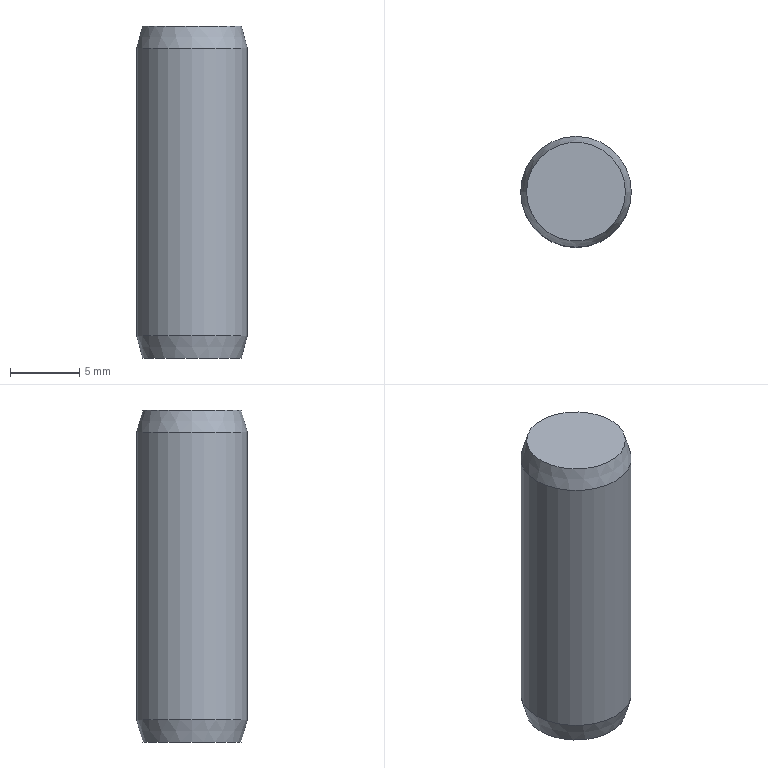Component | NX | GB-T119_1-2000_8X24 | 1 solid | 5 faces | box 8 x 8 x 24 mm | volume 1190 mm3 | plane 2 | cone 2 | cylinder 1 | commonest cylinder face diameters 8 x1
STEP:
#1=CARTESIAN_POINT('',(0.,0.,0.));
#2=DIRECTION('',(0.,0.,1.));
#3=DIRECTION('',(1.,0.,0.));
#4=AXIS2_PLACEMENT_3D('',#1,#2,#3);
#5=CARTESIAN_POINT('',(86.429,-75.,-100.));
#6=VERTEX_POINT('',#5);
#7=CARTESIAN_POINT('',(90.,-75.,-100.));
#8=DIRECTION('',(0.,0.,-1.));
#9=DIRECTION('',(-1.,0.,0.));
#10=AXIS2_PLACEMENT_3D('',#7,#8,#9);
#11=CIRCLE('',#10,3.571);
#12=CARTESIAN_POINT('',(90.,-75.,-100.));
#13=DIRECTION('',(0.,0.,-1.));
#14=DIRECTION('',(-1.,0.,0.));
#15=AXIS2_PLACEMENT_3D('',#12,#13,#14);
#16=PLANE('',#15);
#17=CARTESIAN_POINT('',(0.,0.));
#18=DIRECTION('',(1.,0.));
#19=AXIS2_PLACEMENT_2D('',#17,#18);
#20=CIRCLE('',#19,3.571);
#21=(GEOMETRIC_REPRESENTATION_CONTEXT(2)PARAMETRIC_REPRESENTATION_CONTEXT()REPRESENTATION_CONTEXT('',''));
#22=DEFINITIONAL_REPRESENTATION('',(#20),#21);
#23=PCURVE('',#16,#22);
#24=CARTESIAN_POINT('',(90.,-75.,-100.));
#25=DIRECTION('',(0.,0.,1.));
#26=DIRECTION('',(1.,0.,0.));
#27=AXIS2_PLACEMENT_3D('',#24,#25,#26);
#28=CONICAL_SURFACE('',#27,3.571,0.2618);
#29=CARTESIAN_POINT('',(9.425,0.));
#30=DIRECTION('',(-1.,0.));
#31=VECTOR('',#30,1.);
#32=LINE('',#29,#31);
#33=(GEOMETRIC_REPRESENTATION_CONTEXT(2)PARAMETRIC_REPRESENTATION_CONTEXT()REPRESENTATION_CONTEXT('',''));
#34=DEFINITIONAL_REPRESENTATION('',(#32),#33);
#35=PCURVE('',#28,#34);
#36=SURFACE_CURVE('',#11,(#23,#35),.PCURVE_S1.);
#37=EDGE_CURVE('',#6,#6,#36,.T.);
#38=ORIENTED_EDGE('',*,*,#37,.T.);
#39=EDGE_LOOP('',(#38));
#40=FACE_BOUND('',#39,.T.);
#41=ADVANCED_FACE('',(#40),#16,.T.);
#42=CARTESIAN_POINT('',(86.,-75.,-98.4));
#43=VERTEX_POINT('',#42);
#44=CARTESIAN_POINT('',(90.,-75.,-98.4));
#45=DIRECTION('',(0.,0.,-1.));
#46=DIRECTION('',(-1.,0.,0.));
#47=AXIS2_PLACEMENT_3D('',#44,#45,#46);
#48=CIRCLE('',#47,4.);
#49=CARTESIAN_POINT('',(9.425,1.6));
#50=DIRECTION('',(-1.,0.));
#51=VECTOR('',#50,1.);
#52=LINE('',#49,#51);
#53=(GEOMETRIC_REPRESENTATION_CONTEXT(2)PARAMETRIC_REPRESENTATION_CONTEXT()REPRESENTATION_CONTEXT('',''));
#54=DEFINITIONAL_REPRESENTATION('',(#52),#53);
#55=PCURVE('',#28,#54);
#56=CARTESIAN_POINT('',(90.,-75.,-76.));
#57=DIRECTION('',(0.,0.,-1.));
#58=DIRECTION('',(-1.,0.,0.));
#59=AXIS2_PLACEMENT_3D('',#56,#57,#58);
#60=CYLINDRICAL_SURFACE('',#59,4.);
#61=CARTESIAN_POINT('',(0.,22.4));
#62=DIRECTION('',(1.,0.));
#63=VECTOR('',#62,1.);
#64=LINE('',#61,#63);
#65=(GEOMETRIC_REPRESENTATION_CONTEXT(2)PARAMETRIC_REPRESENTATION_CONTEXT()REPRESENTATION_CONTEXT('',''));
#66=DEFINITIONAL_REPRESENTATION('',(#64),#65);
#67=PCURVE('',#60,#66);
#68=SURFACE_CURVE('',#48,(#55,#67),.PCURVE_S1.);
#69=EDGE_CURVE('',#43,#43,#68,.T.);
#70=ORIENTED_EDGE('',*,*,#69,.T.);
#71=CARTESIAN_POINT('',(86.429,-75.,-100.));
#72=CARTESIAN_POINT('',(86.,-75.,-98.4));
#73=B_SPLINE_CURVE_WITH_KNOTS('',1,(#71,#72),.UNSPECIFIED.,.F.,.F.,(2,2),(0.,1.656),.PIECEWISE_BEZIER_KNOTS.);
#74=CARTESIAN_POINT('',(3.142,0.));
#75=DIRECTION('',(0.,1.));
#76=VECTOR('',#75,1.);
#77=LINE('',#74,#76);
#78=(GEOMETRIC_REPRESENTATION_CONTEXT(2)PARAMETRIC_REPRESENTATION_CONTEXT()REPRESENTATION_CONTEXT('',''));
#79=DEFINITIONAL_REPRESENTATION('',(#77),#78);
#80=PCURVE('',#28,#79);
#81=CARTESIAN_POINT('',(9.425,0.));
#82=DIRECTION('',(0.,1.));
#83=VECTOR('',#82,1.);
#84=LINE('',#81,#83);
#85=(GEOMETRIC_REPRESENTATION_CONTEXT(2)PARAMETRIC_REPRESENTATION_CONTEXT()REPRESENTATION_CONTEXT('',''));
#86=DEFINITIONAL_REPRESENTATION('',(#84),#85);
#87=PCURVE('',#28,#86);
#88=SEAM_CURVE('',#73,(#80,#87),.PCURVE_S1.);
#89=EDGE_CURVE('',#6,#43,#88,.T.);
#90=ORIENTED_EDGE('',*,*,#89,.F.);
#91=ORIENTED_EDGE('',*,*,#37,.F.);
#92=ORIENTED_EDGE('',*,*,#89,.T.);
#93=EDGE_LOOP('',(#70,#90,#91,#92));
#94=FACE_BOUND('',#93,.T.);
#95=ADVANCED_FACE('',(#94),#28,.T.);
#96=CARTESIAN_POINT('',(86.,-75.,-77.6));
#97=VERTEX_POINT('',#96);
#98=CARTESIAN_POINT('',(90.,-75.,-77.6));
#99=DIRECTION('',(0.,0.,-1.));
#100=DIRECTION('',(-1.,0.,0.));
#101=AXIS2_PLACEMENT_3D('',#98,#99,#100);
#102=CIRCLE('',#101,4.);
#103=CARTESIAN_POINT('',(0.,1.6));
#104=DIRECTION('',(1.,0.));
#105=VECTOR('',#104,1.);
#106=LINE('',#103,#105);
#107=(GEOMETRIC_REPRESENTATION_CONTEXT(2)PARAMETRIC_REPRESENTATION_CONTEXT()REPRESENTATION_CONTEXT('',''));
#108=DEFINITIONAL_REPRESENTATION('',(#106),#107);
#109=PCURVE('',#60,#108);
#110=CARTESIAN_POINT('',(90.,-75.,-77.6));
#111=DIRECTION('',(0.,0.,-1.));
#112=DIRECTION('',(-1.,0.,0.));
#113=AXIS2_PLACEMENT_3D('',#110,#111,#112);
#114=CONICAL_SURFACE('',#113,4.,0.2618);
#115=CARTESIAN_POINT('',(0.,0.));
#116=DIRECTION('',(1.,0.));
#117=VECTOR('',#116,1.);
#118=LINE('',#115,#117);
#119=(GEOMETRIC_REPRESENTATION_CONTEXT(2)PARAMETRIC_REPRESENTATION_CONTEXT()REPRESENTATION_CONTEXT('',''));
#120=DEFINITIONAL_REPRESENTATION('',(#118),#119);
#121=PCURVE('',#114,#120);
#122=SURFACE_CURVE('',#102,(#109,#121),.PCURVE_S1.);
#123=EDGE_CURVE('',#97,#97,#122,.T.);
#124=ORIENTED_EDGE('',*,*,#123,.T.);
#125=CARTESIAN_POINT('',(86.,-75.,-77.6));
#126=CARTESIAN_POINT('',(86.,-75.,-98.4));
#127=B_SPLINE_CURVE_WITH_KNOTS('',1,(#125,#126),.UNSPECIFIED.,.F.,.F.,(2,2),(1.6,22.4),.PIECEWISE_BEZIER_KNOTS.);
#128=CARTESIAN_POINT('',(6.283,0.));
#129=DIRECTION('',(0.,1.));
#130=VECTOR('',#129,1.);
#131=LINE('',#128,#130);
#132=(GEOMETRIC_REPRESENTATION_CONTEXT(2)PARAMETRIC_REPRESENTATION_CONTEXT()REPRESENTATION_CONTEXT('',''));
#133=DEFINITIONAL_REPRESENTATION('',(#131),#132);
#134=PCURVE('',#60,#133);
#135=CARTESIAN_POINT('',(0.,0.));
#136=DIRECTION('',(0.,1.));
#137=VECTOR('',#136,1.);
#138=LINE('',#135,#137);
#139=(GEOMETRIC_REPRESENTATION_CONTEXT(2)PARAMETRIC_REPRESENTATION_CONTEXT()REPRESENTATION_CONTEXT('',''));
#140=DEFINITIONAL_REPRESENTATION('',(#138),#139);
#141=PCURVE('',#60,#140);
#142=SEAM_CURVE('',#127,(#134,#141),.PCURVE_S1.);
#143=EDGE_CURVE('',#97,#43,#142,.T.);
#144=ORIENTED_EDGE('',*,*,#143,.T.);
#145=ORIENTED_EDGE('',*,*,#69,.F.);
#146=ORIENTED_EDGE('',*,*,#143,.F.);
#147=EDGE_LOOP('',(#124,#144,#145,#146));
#148=FACE_BOUND('',#147,.T.);
#149=ADVANCED_FACE('',(#148),#60,.T.);
#150=CARTESIAN_POINT('',(86.429,-75.,-76.));
#151=VERTEX_POINT('',#150);
#152=CARTESIAN_POINT('',(90.,-75.,-76.));
#153=DIRECTION('',(0.,0.,-1.));
#154=DIRECTION('',(-1.,0.,0.));
#155=AXIS2_PLACEMENT_3D('',#152,#153,#154);
#156=CIRCLE('',#155,3.571);
#157=CARTESIAN_POINT('',(0.,-1.6));
#158=DIRECTION('',(1.,0.));
#159=VECTOR('',#158,1.);
#160=LINE('',#157,#159);
#161=(GEOMETRIC_REPRESENTATION_CONTEXT(2)PARAMETRIC_REPRESENTATION_CONTEXT()REPRESENTATION_CONTEXT('',''));
#162=DEFINITIONAL_REPRESENTATION('',(#160),#161);
#163=PCURVE('',#114,#162);
#164=CARTESIAN_POINT('',(93.571,-75.,-76.));
#165=DIRECTION('',(0.,0.,1.));
#166=DIRECTION('',(1.,0.,0.));
#167=AXIS2_PLACEMENT_3D('',#164,#165,#166);
#168=PLANE('',#167);
#169=CARTESIAN_POINT('',(-7.143,0.));
#170=CARTESIAN_POINT('',(-7.143,6.186));
#171=CARTESIAN_POINT('',(-1.786,3.093));
#172=CARTESIAN_POINT('',(3.571,0.));
#173=CARTESIAN_POINT('',(-1.786,-3.093));
#174=CARTESIAN_POINT('',(-7.143,-6.186));
#175=CARTESIAN_POINT('',(-7.143,0.));
#176=(BOUNDED_CURVE()B_SPLINE_CURVE(2,(#169,#170,#171,#172,#173,#174,#175),.UNSPECIFIED.,.T.,.F.)B_SPLINE_CURVE_WITH_KNOTS((1,2,2,2,2,1),(-2.094,0.,2.094,4.189,6.283,8.378),.UNSPECIFIED.)CURVE()GEOMETRIC_REPRESENTATION_ITEM()RATIONAL_B_SPLINE_CURVE((1.,0.5,1.,0.5,1.,0.5,1.))REPRESENTATION_ITEM(''));
#177=(GEOMETRIC_REPRESENTATION_CONTEXT(2)PARAMETRIC_REPRESENTATION_CONTEXT()REPRESENTATION_CONTEXT('',''));
#178=DEFINITIONAL_REPRESENTATION('',(#176),#177);
#179=PCURVE('',#168,#178);
#180=SURFACE_CURVE('',#156,(#163,#179),.PCURVE_S1.);
#181=EDGE_CURVE('',#151,#151,#180,.T.);
#182=ORIENTED_EDGE('',*,*,#181,.T.);
#183=CARTESIAN_POINT('',(86.429,-75.,-76.));
#184=CARTESIAN_POINT('',(86.,-75.,-77.6));
#185=B_SPLINE_CURVE_WITH_KNOTS('',1,(#183,#184),.UNSPECIFIED.,.F.,.F.,(2,2),(-1.656,0.),.PIECEWISE_BEZIER_KNOTS.);
#186=CARTESIAN_POINT('',(6.283,0.));
#187=DIRECTION('',(0.,1.));
#188=VECTOR('',#187,1.);
#189=LINE('',#186,#188);
#190=(GEOMETRIC_REPRESENTATION_CONTEXT(2)PARAMETRIC_REPRESENTATION_CONTEXT()REPRESENTATION_CONTEXT('',''));
#191=DEFINITIONAL_REPRESENTATION('',(#189),#190);
#192=PCURVE('',#114,#191);
#193=CARTESIAN_POINT('',(0.,0.));
#194=DIRECTION('',(0.,1.));
#195=VECTOR('',#194,1.);
#196=LINE('',#193,#195);
#197=(GEOMETRIC_REPRESENTATION_CONTEXT(2)PARAMETRIC_REPRESENTATION_CONTEXT()REPRESENTATION_CONTEXT('',''));
#198=DEFINITIONAL_REPRESENTATION('',(#196),#197);
#199=PCURVE('',#114,#198);
#200=SEAM_CURVE('',#185,(#192,#199),.PCURVE_S1.);
#201=EDGE_CURVE('',#151,#97,#200,.T.);
#202=ORIENTED_EDGE('',*,*,#201,.T.);
#203=ORIENTED_EDGE('',*,*,#123,.F.);
#204=ORIENTED_EDGE('',*,*,#201,.F.);
#205=EDGE_LOOP('',(#182,#202,#203,#204));
#206=FACE_BOUND('',#205,.T.);
#207=ADVANCED_FACE('',(#206),#114,.T.);
#208=ORIENTED_EDGE('',*,*,#181,.F.);
#209=EDGE_LOOP('',(#208));
#210=FACE_BOUND('',#209,.T.);
#211=ADVANCED_FACE('',(#210),#168,.T.);
#212=CLOSED_SHELL('',(#41,#95,#149,#207,#211));
#213=MANIFOLD_SOLID_BREP('',#212);
#214=(LENGTH_UNIT()NAMED_UNIT(*)SI_UNIT(.MILLI.,.METRE.));
#215=UNCERTAINTY_MEASURE_WITH_UNIT(LENGTH_MEASURE(0.00001),#214,'','');
#216=(NAMED_UNIT(*)PLANE_ANGLE_UNIT()SI_UNIT($,.RADIAN.));
#217=(NAMED_UNIT(*)SI_UNIT($,.STERADIAN.)SOLID_ANGLE_UNIT());
#218=(GEOMETRIC_REPRESENTATION_CONTEXT(3)GLOBAL_UNCERTAINTY_ASSIGNED_CONTEXT((#215))GLOBAL_UNIT_ASSIGNED_CONTEXT((#214,#216,#217))REPRESENTATION_CONTEXT('',''));
#219=ADVANCED_BREP_SHAPE_REPRESENTATION('',(#4,#213),#218);